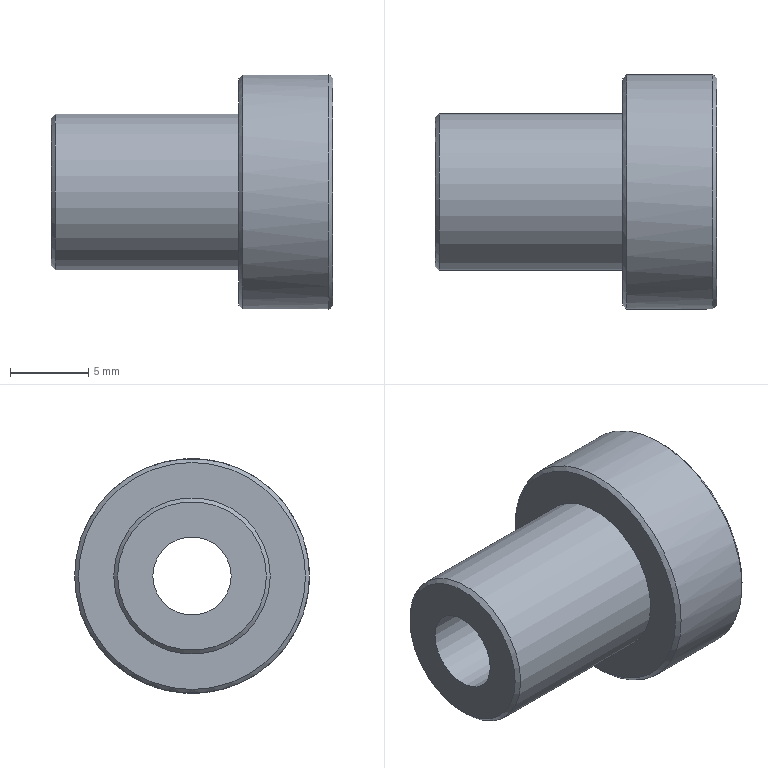Component | NX | PORT_1_2 | 1 solid | 9 faces | box 18 x 15 x 15 mm | volume 1645 mm3 | plane 3 | cylinder 3 | cone 3 | commonest cylinder face diameters 10 x1 15 x1 5 x1
STEP:
#1=CARTESIAN_POINT('',(0.,0.,0.));
#2=DIRECTION('',(0.,0.,1.));
#3=DIRECTION('',(1.,0.,0.));
#4=AXIS2_PLACEMENT_3D('',#1,#2,#3);
#5=CARTESIAN_POINT('',(-69.,-39.25,41.));
#6=VERTEX_POINT('',#5);
#7=CARTESIAN_POINT('',(-69.,-34.25,41.));
#8=VERTEX_POINT('',#7);
#9=CARTESIAN_POINT('',(-69.,-36.75,41.));
#10=DIRECTION('',(1.,0.,0.));
#11=DIRECTION('',(0.,-1.,0.));
#12=AXIS2_PLACEMENT_3D('',#9,#10,#11);
#13=CIRCLE('',#12,2.5);
#14=CARTESIAN_POINT('',(-69.,-36.75,41.));
#15=DIRECTION('',(-1.,0.,0.));
#16=DIRECTION('',(0.,-1.,0.));
#17=AXIS2_PLACEMENT_3D('',#14,#15,#16);
#18=PLANE('',#17);
#19=CARTESIAN_POINT('',(2.5,0.));
#20=CARTESIAN_POINT('',(2.5,-4.33));
#21=CARTESIAN_POINT('',(-1.25,-2.165));
#22=CARTESIAN_POINT('',(-5.,-0.));
#23=CARTESIAN_POINT('',(-1.25,2.165));
#24=CARTESIAN_POINT('',(2.5,4.33));
#25=CARTESIAN_POINT('',(2.5,0.));
#26=(BOUNDED_CURVE()B_SPLINE_CURVE(2,(#19,#20,#21,#22,#23,#24,#25),.UNSPECIFIED.,.T.,.F.)B_SPLINE_CURVE_WITH_KNOTS((1,2,2,2,2,1),(-2.094,0.,2.094,4.189,6.283,8.378),.UNSPECIFIED.)CURVE()GEOMETRIC_REPRESENTATION_ITEM()RATIONAL_B_SPLINE_CURVE((1.,0.5,1.,0.5,1.,0.5,1.))REPRESENTATION_ITEM(''));
#27=(GEOMETRIC_REPRESENTATION_CONTEXT(2)PARAMETRIC_REPRESENTATION_CONTEXT()REPRESENTATION_CONTEXT('',''));
#28=DEFINITIONAL_REPRESENTATION('',(#26),#27);
#29=PCURVE('',#18,#28);
#30=CARTESIAN_POINT('',(-76.,-36.75,41.));
#31=DIRECTION('',(1.,0.,0.));
#32=DIRECTION('',(0.,1.,0.));
#33=AXIS2_PLACEMENT_3D('',#30,#31,#32);
#34=CYLINDRICAL_SURFACE('',#33,2.5);
#35=CARTESIAN_POINT('',(3.142,7.));
#36=DIRECTION('',(1.,0.));
#37=VECTOR('',#36,1.);
#38=LINE('',#35,#37);
#39=(GEOMETRIC_REPRESENTATION_CONTEXT(2)PARAMETRIC_REPRESENTATION_CONTEXT()REPRESENTATION_CONTEXT('',''));
#40=DEFINITIONAL_REPRESENTATION('',(#38),#39);
#41=PCURVE('',#34,#40);
#42=SURFACE_CURVE('',#13,(#29,#41),.PCURVE_S1.);
#43=EDGE_CURVE('',#6,#8,#42,.T.);
#44=ORIENTED_EDGE('',*,*,#43,.T.);
#45=CARTESIAN_POINT('',(-69.,-36.75,41.));
#46=DIRECTION('',(1.,0.,0.));
#47=DIRECTION('',(0.,-1.,0.));
#48=AXIS2_PLACEMENT_3D('',#45,#46,#47);
#49=CIRCLE('',#48,2.5);
#50=CARTESIAN_POINT('',(2.5,0.));
#51=CARTESIAN_POINT('',(2.5,-4.33));
#52=CARTESIAN_POINT('',(-1.25,-2.165));
#53=CARTESIAN_POINT('',(-5.,-0.));
#54=CARTESIAN_POINT('',(-1.25,2.165));
#55=CARTESIAN_POINT('',(2.5,4.33));
#56=CARTESIAN_POINT('',(2.5,0.));
#57=(BOUNDED_CURVE()B_SPLINE_CURVE(2,(#50,#51,#52,#53,#54,#55,#56),.UNSPECIFIED.,.T.,.F.)B_SPLINE_CURVE_WITH_KNOTS((1,2,2,2,2,1),(-2.094,0.,2.094,4.189,6.283,8.378),.UNSPECIFIED.)CURVE()GEOMETRIC_REPRESENTATION_ITEM()RATIONAL_B_SPLINE_CURVE((1.,0.5,1.,0.5,1.,0.5,1.))REPRESENTATION_ITEM(''));
#58=(GEOMETRIC_REPRESENTATION_CONTEXT(2)PARAMETRIC_REPRESENTATION_CONTEXT()REPRESENTATION_CONTEXT('',''));
#59=DEFINITIONAL_REPRESENTATION('',(#57),#58);
#60=PCURVE('',#18,#59);
#61=CARTESIAN_POINT('',(-3.142,7.));
#62=DIRECTION('',(1.,0.));
#63=VECTOR('',#62,1.);
#64=LINE('',#61,#63);
#65=(GEOMETRIC_REPRESENTATION_CONTEXT(2)PARAMETRIC_REPRESENTATION_CONTEXT()REPRESENTATION_CONTEXT('',''));
#66=DEFINITIONAL_REPRESENTATION('',(#64),#65);
#67=PCURVE('',#34,#66);
#68=SURFACE_CURVE('',#49,(#60,#67),.PCURVE_S1.);
#69=EDGE_CURVE('',#8,#6,#68,.T.);
#70=ORIENTED_EDGE('',*,*,#69,.T.);
#71=EDGE_LOOP('',(#44,#70));
#72=FACE_BOUND('',#71,.T.);
#73=CARTESIAN_POINT('',(-69.,-41.5,41.));
#74=VERTEX_POINT('',#73);
#75=CARTESIAN_POINT('',(-69.,-36.75,41.));
#76=DIRECTION('',(-1.,0.,0.));
#77=DIRECTION('',(0.,-1.,0.));
#78=AXIS2_PLACEMENT_3D('',#75,#76,#77);
#79=CIRCLE('',#78,4.75);
#80=CARTESIAN_POINT('',(0.,0.));
#81=DIRECTION('',(1.,0.));
#82=AXIS2_PLACEMENT_2D('',#80,#81);
#83=CIRCLE('',#82,4.75);
#84=(GEOMETRIC_REPRESENTATION_CONTEXT(2)PARAMETRIC_REPRESENTATION_CONTEXT()REPRESENTATION_CONTEXT('',''));
#85=DEFINITIONAL_REPRESENTATION('',(#83),#84);
#86=PCURVE('',#18,#85);
#87=CARTESIAN_POINT('',(-68.75,-36.75,41.));
#88=DIRECTION('',(1.,0.,0.));
#89=DIRECTION('',(0.,1.,0.));
#90=AXIS2_PLACEMENT_3D('',#87,#88,#89);
#91=CONICAL_SURFACE('',#90,5.,0.7854);
#92=CARTESIAN_POINT('',(9.425,-0.25));
#93=DIRECTION('',(-1.,0.));
#94=VECTOR('',#93,1.);
#95=LINE('',#92,#94);
#96=(GEOMETRIC_REPRESENTATION_CONTEXT(2)PARAMETRIC_REPRESENTATION_CONTEXT()REPRESENTATION_CONTEXT('',''));
#97=DEFINITIONAL_REPRESENTATION('',(#95),#96);
#98=PCURVE('',#91,#97);
#99=SURFACE_CURVE('',#79,(#86,#98),.PCURVE_S1.);
#100=EDGE_CURVE('',#74,#74,#99,.T.);
#101=ORIENTED_EDGE('',*,*,#100,.T.);
#102=EDGE_LOOP('',(#101));
#103=FACE_BOUND('',#102,.T.);
#104=ADVANCED_FACE('',(#72,#103),#18,.T.);
#105=CARTESIAN_POINT('',(-68.75,-41.75,41.));
#106=VERTEX_POINT('',#105);
#107=CARTESIAN_POINT('',(-68.75,-31.75,41.));
#108=VERTEX_POINT('',#107);
#109=CARTESIAN_POINT('',(-68.75,-36.75,41.));
#110=DIRECTION('',(1.,0.,0.));
#111=DIRECTION('',(0.,-1.,0.));
#112=AXIS2_PLACEMENT_3D('',#109,#110,#111);
#113=CIRCLE('',#112,5.);
#114=CARTESIAN_POINT('',(-69.,-36.75,41.));
#115=DIRECTION('',(1.,0.,0.));
#116=DIRECTION('',(0.,1.,0.));
#117=AXIS2_PLACEMENT_3D('',#114,#115,#116);
#118=CYLINDRICAL_SURFACE('',#117,5.);
#119=CARTESIAN_POINT('',(3.142,0.25));
#120=DIRECTION('',(1.,0.));
#121=VECTOR('',#120,1.);
#122=LINE('',#119,#121);
#123=(GEOMETRIC_REPRESENTATION_CONTEXT(2)PARAMETRIC_REPRESENTATION_CONTEXT()REPRESENTATION_CONTEXT('',''));
#124=DEFINITIONAL_REPRESENTATION('',(#122),#123);
#125=PCURVE('',#118,#124);
#126=CARTESIAN_POINT('',(3.142,0.));
#127=DIRECTION('',(1.,0.));
#128=VECTOR('',#127,1.);
#129=LINE('',#126,#128);
#130=(GEOMETRIC_REPRESENTATION_CONTEXT(2)PARAMETRIC_REPRESENTATION_CONTEXT()REPRESENTATION_CONTEXT('',''));
#131=DEFINITIONAL_REPRESENTATION('',(#129),#130);
#132=PCURVE('',#91,#131);
#133=SURFACE_CURVE('',#113,(#125,#132),.PCURVE_S1.);
#134=EDGE_CURVE('',#106,#108,#133,.T.);
#135=ORIENTED_EDGE('',*,*,#134,.T.);
#136=CARTESIAN_POINT('',(-57.,-31.75,41.));
#137=VERTEX_POINT('',#136);
#138=CARTESIAN_POINT('',(-68.75,-31.75,41.));
#139=CARTESIAN_POINT('',(-57.,-31.75,41.));
#140=B_SPLINE_CURVE_WITH_KNOTS('',1,(#138,#139),.UNSPECIFIED.,.F.,.F.,(2,2),(0.25,12.),.PIECEWISE_BEZIER_KNOTS.);
#141=CARTESIAN_POINT('',(6.283,0.));
#142=DIRECTION('',(0.,1.));
#143=VECTOR('',#142,1.);
#144=LINE('',#141,#143);
#145=(GEOMETRIC_REPRESENTATION_CONTEXT(2)PARAMETRIC_REPRESENTATION_CONTEXT()REPRESENTATION_CONTEXT('',''));
#146=DEFINITIONAL_REPRESENTATION('',(#144),#145);
#147=PCURVE('',#118,#146);
#148=CARTESIAN_POINT('',(0.,0.));
#149=DIRECTION('',(0.,1.));
#150=VECTOR('',#149,1.);
#151=LINE('',#148,#150);
#152=(GEOMETRIC_REPRESENTATION_CONTEXT(2)PARAMETRIC_REPRESENTATION_CONTEXT()REPRESENTATION_CONTEXT('',''));
#153=DEFINITIONAL_REPRESENTATION('',(#151),#152);
#154=PCURVE('',#118,#153);
#155=SEAM_CURVE('',#140,(#147,#154),.PCURVE_S1.);
#156=EDGE_CURVE('',#108,#137,#155,.T.);
#157=ORIENTED_EDGE('',*,*,#156,.T.);
#158=CARTESIAN_POINT('',(-57.,-36.75,41.));
#159=DIRECTION('',(-1.,0.,0.));
#160=DIRECTION('',(0.,1.,0.));
#161=AXIS2_PLACEMENT_3D('',#158,#159,#160);
#162=CIRCLE('',#161,5.);
#163=CARTESIAN_POINT('',(6.283,12.));
#164=DIRECTION('',(-1.,0.));
#165=VECTOR('',#164,1.);
#166=LINE('',#163,#165);
#167=(GEOMETRIC_REPRESENTATION_CONTEXT(2)PARAMETRIC_REPRESENTATION_CONTEXT()REPRESENTATION_CONTEXT('',''));
#168=DEFINITIONAL_REPRESENTATION('',(#166),#167);
#169=PCURVE('',#118,#168);
#170=CARTESIAN_POINT('',(-57.,-36.75,41.));
#171=DIRECTION('',(-1.,0.,0.));
#172=DIRECTION('',(0.,-1.,0.));
#173=AXIS2_PLACEMENT_3D('',#170,#171,#172);
#174=PLANE('',#173);
#175=CARTESIAN_POINT('',(0.,0.));
#176=DIRECTION('',(-1.,0.));
#177=AXIS2_PLACEMENT_2D('',#175,#176);
#178=CIRCLE('',#177,5.);
#179=(GEOMETRIC_REPRESENTATION_CONTEXT(2)PARAMETRIC_REPRESENTATION_CONTEXT()REPRESENTATION_CONTEXT('',''));
#180=DEFINITIONAL_REPRESENTATION('',(#178),#179);
#181=PCURVE('',#174,#180);
#182=SURFACE_CURVE('',#162,(#169,#181),.PCURVE_S1.);
#183=EDGE_CURVE('',#137,#137,#182,.T.);
#184=ORIENTED_EDGE('',*,*,#183,.T.);
#185=ORIENTED_EDGE('',*,*,#156,.F.);
#186=CARTESIAN_POINT('',(-68.75,-36.75,41.));
#187=DIRECTION('',(1.,0.,0.));
#188=DIRECTION('',(0.,-1.,0.));
#189=AXIS2_PLACEMENT_3D('',#186,#187,#188);
#190=CIRCLE('',#189,5.);
#191=CARTESIAN_POINT('',(-3.142,0.25));
#192=DIRECTION('',(1.,0.));
#193=VECTOR('',#192,1.);
#194=LINE('',#191,#193);
#195=(GEOMETRIC_REPRESENTATION_CONTEXT(2)PARAMETRIC_REPRESENTATION_CONTEXT()REPRESENTATION_CONTEXT('',''));
#196=DEFINITIONAL_REPRESENTATION('',(#194),#195);
#197=PCURVE('',#118,#196);
#198=CARTESIAN_POINT('',(3.142,0.));
#199=DIRECTION('',(1.,0.));
#200=VECTOR('',#199,1.);
#201=LINE('',#198,#200);
#202=(GEOMETRIC_REPRESENTATION_CONTEXT(2)PARAMETRIC_REPRESENTATION_CONTEXT()REPRESENTATION_CONTEXT('',''));
#203=DEFINITIONAL_REPRESENTATION('',(#201),#202);
#204=PCURVE('',#91,#203);
#205=SURFACE_CURVE('',#190,(#197,#204),.PCURVE_S1.);
#206=EDGE_CURVE('',#108,#106,#205,.T.);
#207=ORIENTED_EDGE('',*,*,#206,.T.);
#208=EDGE_LOOP('',(#135,#157,#184,#185,#207));
#209=FACE_BOUND('',#208,.T.);
#210=ADVANCED_FACE('',(#209),#118,.T.);
#211=CARTESIAN_POINT('',(-51.,-34.25,41.));
#212=VERTEX_POINT('',#211);
#213=CARTESIAN_POINT('',(-51.,-36.75,41.));
#214=DIRECTION('',(-1.,0.,0.));
#215=DIRECTION('',(0.,1.,0.));
#216=AXIS2_PLACEMENT_3D('',#213,#214,#215);
#217=CIRCLE('',#216,2.5);
#218=CARTESIAN_POINT('',(-51.,-36.75,41.));
#219=DIRECTION('',(1.,0.,0.));
#220=DIRECTION('',(0.,1.,0.));
#221=AXIS2_PLACEMENT_3D('',#218,#219,#220);
#222=PLANE('',#221);
#223=CARTESIAN_POINT('',(2.5,0.));
#224=CARTESIAN_POINT('',(2.5,-4.33));
#225=CARTESIAN_POINT('',(-1.25,-2.165));
#226=CARTESIAN_POINT('',(-5.,-0.));
#227=CARTESIAN_POINT('',(-1.25,2.165));
#228=CARTESIAN_POINT('',(2.5,4.33));
#229=CARTESIAN_POINT('',(2.5,0.));
#230=(BOUNDED_CURVE()B_SPLINE_CURVE(2,(#223,#224,#225,#226,#227,#228,#229),.UNSPECIFIED.,.T.,.F.)B_SPLINE_CURVE_WITH_KNOTS((1,2,2,2,2,1),(-2.094,0.,2.094,4.189,6.283,8.378),.UNSPECIFIED.)CURVE()GEOMETRIC_REPRESENTATION_ITEM()RATIONAL_B_SPLINE_CURVE((1.,0.5,1.,0.5,1.,0.5,1.))REPRESENTATION_ITEM(''));
#231=(GEOMETRIC_REPRESENTATION_CONTEXT(2)PARAMETRIC_REPRESENTATION_CONTEXT()REPRESENTATION_CONTEXT('',''));
#232=DEFINITIONAL_REPRESENTATION('',(#230),#231);
#233=PCURVE('',#222,#232);
#234=CARTESIAN_POINT('',(6.283,25.));
#235=DIRECTION('',(-1.,0.));
#236=VECTOR('',#235,1.);
#237=LINE('',#234,#236);
#238=(GEOMETRIC_REPRESENTATION_CONTEXT(2)PARAMETRIC_REPRESENTATION_CONTEXT()REPRESENTATION_CONTEXT('',''));
#239=DEFINITIONAL_REPRESENTATION('',(#237),#238);
#240=PCURVE('',#34,#239);
#241=SURFACE_CURVE('',#217,(#233,#240),.PCURVE_S1.);
#242=EDGE_CURVE('',#212,#212,#241,.T.);
#243=ORIENTED_EDGE('',*,*,#242,.T.);
#244=EDGE_LOOP('',(#243));
#245=FACE_BOUND('',#244,.T.);
#246=CARTESIAN_POINT('',(-51.,-29.5,41.));
#247=VERTEX_POINT('',#246);
#248=CARTESIAN_POINT('',(-51.,-36.75,41.));
#249=DIRECTION('',(1.,0.,0.));
#250=DIRECTION('',(0.,1.,0.));
#251=AXIS2_PLACEMENT_3D('',#248,#249,#250);
#252=CIRCLE('',#251,7.25);
#253=CARTESIAN_POINT('',(0.,0.));
#254=DIRECTION('',(1.,0.));
#255=AXIS2_PLACEMENT_2D('',#253,#254);
#256=CIRCLE('',#255,7.25);
#257=(GEOMETRIC_REPRESENTATION_CONTEXT(2)PARAMETRIC_REPRESENTATION_CONTEXT()REPRESENTATION_CONTEXT('',''));
#258=DEFINITIONAL_REPRESENTATION('',(#256),#257);
#259=PCURVE('',#222,#258);
#260=CARTESIAN_POINT('',(-51.,-36.75,41.));
#261=DIRECTION('',(-1.,0.,0.));
#262=DIRECTION('',(0.,-1.,0.));
#263=AXIS2_PLACEMENT_3D('',#260,#261,#262);
#264=CONICAL_SURFACE('',#263,7.25,0.7854);
#265=CARTESIAN_POINT('',(9.425,0.));
#266=DIRECTION('',(-1.,0.));
#267=VECTOR('',#266,1.);
#268=LINE('',#265,#267);
#269=(GEOMETRIC_REPRESENTATION_CONTEXT(2)PARAMETRIC_REPRESENTATION_CONTEXT()REPRESENTATION_CONTEXT('',''));
#270=DEFINITIONAL_REPRESENTATION('',(#268),#269);
#271=PCURVE('',#264,#270);
#272=SURFACE_CURVE('',#252,(#259,#271),.PCURVE_S1.);
#273=EDGE_CURVE('',#247,#247,#272,.T.);
#274=ORIENTED_EDGE('',*,*,#273,.T.);
#275=EDGE_LOOP('',(#274));
#276=FACE_BOUND('',#275,.T.);
#277=ADVANCED_FACE('',(#245,#276),#222,.T.);
#278=CARTESIAN_POINT('',(-57.,-44.,41.));
#279=VERTEX_POINT('',#278);
#280=CARTESIAN_POINT('',(-57.,-36.75,41.));
#281=DIRECTION('',(-1.,0.,0.));
#282=DIRECTION('',(0.,-1.,0.));
#283=AXIS2_PLACEMENT_3D('',#280,#281,#282);
#284=CIRCLE('',#283,7.25);
#285=CARTESIAN_POINT('',(0.,0.));
#286=DIRECTION('',(1.,0.));
#287=AXIS2_PLACEMENT_2D('',#285,#286);
#288=CIRCLE('',#287,7.25);
#289=(GEOMETRIC_REPRESENTATION_CONTEXT(2)PARAMETRIC_REPRESENTATION_CONTEXT()REPRESENTATION_CONTEXT('',''));
#290=DEFINITIONAL_REPRESENTATION('',(#288),#289);
#291=PCURVE('',#174,#290);
#292=CARTESIAN_POINT('',(-56.75,-36.75,41.));
#293=DIRECTION('',(1.,0.,0.));
#294=DIRECTION('',(0.,1.,0.));
#295=AXIS2_PLACEMENT_3D('',#292,#293,#294);
#296=CONICAL_SURFACE('',#295,7.5,0.7854);
#297=CARTESIAN_POINT('',(9.425,-0.25));
#298=DIRECTION('',(-1.,0.));
#299=VECTOR('',#298,1.);
#300=LINE('',#297,#299);
#301=(GEOMETRIC_REPRESENTATION_CONTEXT(2)PARAMETRIC_REPRESENTATION_CONTEXT()REPRESENTATION_CONTEXT('',''));
#302=DEFINITIONAL_REPRESENTATION('',(#300),#301);
#303=PCURVE('',#296,#302);
#304=SURFACE_CURVE('',#284,(#291,#303),.PCURVE_S1.);
#305=EDGE_CURVE('',#279,#279,#304,.T.);
#306=ORIENTED_EDGE('',*,*,#305,.T.);
#307=EDGE_LOOP('',(#306));
#308=FACE_BOUND('',#307,.T.);
#309=ORIENTED_EDGE('',*,*,#183,.F.);
#310=EDGE_LOOP('',(#309));
#311=FACE_BOUND('',#310,.T.);
#312=ADVANCED_FACE('',(#308,#311),#174,.T.);
#313=CARTESIAN_POINT('',(-56.75,-44.25,41.));
#314=VERTEX_POINT('',#313);
#315=CARTESIAN_POINT('',(-56.75,-29.25,41.));
#316=VERTEX_POINT('',#315);
#317=CARTESIAN_POINT('',(-56.75,-36.75,41.));
#318=DIRECTION('',(1.,0.,0.));
#319=DIRECTION('',(0.,-1.,0.));
#320=AXIS2_PLACEMENT_3D('',#317,#318,#319);
#321=CIRCLE('',#320,7.5);
#322=CARTESIAN_POINT('',(-57.,-36.75,41.));
#323=DIRECTION('',(1.,0.,0.));
#324=DIRECTION('',(0.,1.,0.));
#325=AXIS2_PLACEMENT_3D('',#322,#323,#324);
#326=CYLINDRICAL_SURFACE('',#325,7.5);
#327=CARTESIAN_POINT('',(3.142,0.25));
#328=DIRECTION('',(1.,0.));
#329=VECTOR('',#328,1.);
#330=LINE('',#327,#329);
#331=(GEOMETRIC_REPRESENTATION_CONTEXT(2)PARAMETRIC_REPRESENTATION_CONTEXT()REPRESENTATION_CONTEXT('',''));
#332=DEFINITIONAL_REPRESENTATION('',(#330),#331);
#333=PCURVE('',#326,#332);
#334=CARTESIAN_POINT('',(3.142,0.));
#335=DIRECTION('',(1.,0.));
#336=VECTOR('',#335,1.);
#337=LINE('',#334,#336);
#338=(GEOMETRIC_REPRESENTATION_CONTEXT(2)PARAMETRIC_REPRESENTATION_CONTEXT()REPRESENTATION_CONTEXT('',''));
#339=DEFINITIONAL_REPRESENTATION('',(#337),#338);
#340=PCURVE('',#296,#339);
#341=SURFACE_CURVE('',#321,(#333,#340),.PCURVE_S1.);
#342=EDGE_CURVE('',#314,#316,#341,.T.);
#343=ORIENTED_EDGE('',*,*,#342,.T.);
#344=CARTESIAN_POINT('',(-51.25,-29.25,41.));
#345=VERTEX_POINT('',#344);
#346=CARTESIAN_POINT('',(-56.75,-29.25,41.));
#347=CARTESIAN_POINT('',(-51.25,-29.25,41.));
#348=B_SPLINE_CURVE_WITH_KNOTS('',1,(#346,#347),.UNSPECIFIED.,.F.,.F.,(2,2),(0.25,5.75),.PIECEWISE_BEZIER_KNOTS.);
#349=CARTESIAN_POINT('',(6.283,0.));
#350=DIRECTION('',(0.,1.));
#351=VECTOR('',#350,1.);
#352=LINE('',#349,#351);
#353=(GEOMETRIC_REPRESENTATION_CONTEXT(2)PARAMETRIC_REPRESENTATION_CONTEXT()REPRESENTATION_CONTEXT('',''));
#354=DEFINITIONAL_REPRESENTATION('',(#352),#353);
#355=PCURVE('',#326,#354);
#356=CARTESIAN_POINT('',(0.,0.));
#357=DIRECTION('',(0.,1.));
#358=VECTOR('',#357,1.);
#359=LINE('',#356,#358);
#360=(GEOMETRIC_REPRESENTATION_CONTEXT(2)PARAMETRIC_REPRESENTATION_CONTEXT()REPRESENTATION_CONTEXT('',''));
#361=DEFINITIONAL_REPRESENTATION('',(#359),#360);
#362=PCURVE('',#326,#361);
#363=SEAM_CURVE('',#348,(#355,#362),.PCURVE_S1.);
#364=EDGE_CURVE('',#316,#345,#363,.T.);
#365=ORIENTED_EDGE('',*,*,#364,.T.);
#366=CARTESIAN_POINT('',(-51.25,-36.75,41.));
#367=DIRECTION('',(-1.,0.,0.));
#368=DIRECTION('',(0.,1.,0.));
#369=AXIS2_PLACEMENT_3D('',#366,#367,#368);
#370=CIRCLE('',#369,7.5);
#371=CARTESIAN_POINT('',(6.283,5.75));
#372=DIRECTION('',(-1.,0.));
#373=VECTOR('',#372,1.);
#374=LINE('',#371,#373);
#375=(GEOMETRIC_REPRESENTATION_CONTEXT(2)PARAMETRIC_REPRESENTATION_CONTEXT()REPRESENTATION_CONTEXT('',''));
#376=DEFINITIONAL_REPRESENTATION('',(#374),#375);
#377=PCURVE('',#326,#376);
#378=CARTESIAN_POINT('',(3.142,0.25));
#379=DIRECTION('',(1.,0.));
#380=VECTOR('',#379,1.);
#381=LINE('',#378,#380);
#382=(GEOMETRIC_REPRESENTATION_CONTEXT(2)PARAMETRIC_REPRESENTATION_CONTEXT()REPRESENTATION_CONTEXT('',''));
#383=DEFINITIONAL_REPRESENTATION('',(#381),#382);
#384=PCURVE('',#264,#383);
#385=SURFACE_CURVE('',#370,(#377,#384),.PCURVE_S1.);
#386=EDGE_CURVE('',#345,#345,#385,.T.);
#387=ORIENTED_EDGE('',*,*,#386,.T.);
#388=ORIENTED_EDGE('',*,*,#364,.F.);
#389=CARTESIAN_POINT('',(-56.75,-36.75,41.));
#390=DIRECTION('',(1.,0.,0.));
#391=DIRECTION('',(0.,-1.,0.));
#392=AXIS2_PLACEMENT_3D('',#389,#390,#391);
#393=CIRCLE('',#392,7.5);
#394=CARTESIAN_POINT('',(-3.142,0.25));
#395=DIRECTION('',(1.,0.));
#396=VECTOR('',#395,1.);
#397=LINE('',#394,#396);
#398=(GEOMETRIC_REPRESENTATION_CONTEXT(2)PARAMETRIC_REPRESENTATION_CONTEXT()REPRESENTATION_CONTEXT('',''));
#399=DEFINITIONAL_REPRESENTATION('',(#397),#398);
#400=PCURVE('',#326,#399);
#401=CARTESIAN_POINT('',(3.142,0.));
#402=DIRECTION('',(1.,0.));
#403=VECTOR('',#402,1.);
#404=LINE('',#401,#403);
#405=(GEOMETRIC_REPRESENTATION_CONTEXT(2)PARAMETRIC_REPRESENTATION_CONTEXT()REPRESENTATION_CONTEXT('',''));
#406=DEFINITIONAL_REPRESENTATION('',(#404),#405);
#407=PCURVE('',#296,#406);
#408=SURFACE_CURVE('',#393,(#400,#407),.PCURVE_S1.);
#409=EDGE_CURVE('',#316,#314,#408,.T.);
#410=ORIENTED_EDGE('',*,*,#409,.T.);
#411=EDGE_LOOP('',(#343,#365,#387,#388,#410));
#412=FACE_BOUND('',#411,.T.);
#413=ADVANCED_FACE('',(#412),#326,.T.);
#414=ORIENTED_EDGE('',*,*,#305,.F.);
#415=CARTESIAN_POINT('',(-57.,-44.,41.));
#416=CARTESIAN_POINT('',(-56.75,-44.25,41.));
#417=B_SPLINE_CURVE_WITH_KNOTS('',1,(#415,#416),.UNSPECIFIED.,.F.,.F.,(2,2),(-0.3536,0.),.PIECEWISE_BEZIER_KNOTS.);
#418=CARTESIAN_POINT('',(9.425,0.));
#419=DIRECTION('',(0.,1.));
#420=VECTOR('',#419,1.);
#421=LINE('',#418,#420);
#422=(GEOMETRIC_REPRESENTATION_CONTEXT(2)PARAMETRIC_REPRESENTATION_CONTEXT()REPRESENTATION_CONTEXT('',''));
#423=DEFINITIONAL_REPRESENTATION('',(#421),#422);
#424=PCURVE('',#296,#423);
#425=CARTESIAN_POINT('',(3.142,0.));
#426=DIRECTION('',(0.,1.));
#427=VECTOR('',#426,1.);
#428=LINE('',#425,#427);
#429=(GEOMETRIC_REPRESENTATION_CONTEXT(2)PARAMETRIC_REPRESENTATION_CONTEXT()REPRESENTATION_CONTEXT('',''));
#430=DEFINITIONAL_REPRESENTATION('',(#428),#429);
#431=PCURVE('',#296,#430);
#432=SEAM_CURVE('',#417,(#424,#431),.PCURVE_S1.);
#433=EDGE_CURVE('',#279,#314,#432,.T.);
#434=ORIENTED_EDGE('',*,*,#433,.T.);
#435=ORIENTED_EDGE('',*,*,#409,.F.);
#436=ORIENTED_EDGE('',*,*,#342,.F.);
#437=ORIENTED_EDGE('',*,*,#433,.F.);
#438=EDGE_LOOP('',(#414,#434,#435,#436,#437));
#439=FACE_BOUND('',#438,.T.);
#440=ADVANCED_FACE('',(#439),#296,.T.);
#441=ORIENTED_EDGE('',*,*,#386,.F.);
#442=CARTESIAN_POINT('',(-51.,-29.5,41.));
#443=CARTESIAN_POINT('',(-51.25,-29.25,41.));
#444=B_SPLINE_CURVE_WITH_KNOTS('',1,(#442,#443),.UNSPECIFIED.,.F.,.F.,(2,2),(0.,0.3536),.PIECEWISE_BEZIER_KNOTS.);
#445=CARTESIAN_POINT('',(3.142,0.));
#446=DIRECTION('',(0.,1.));
#447=VECTOR('',#446,1.);
#448=LINE('',#445,#447);
#449=(GEOMETRIC_REPRESENTATION_CONTEXT(2)PARAMETRIC_REPRESENTATION_CONTEXT()REPRESENTATION_CONTEXT('',''));
#450=DEFINITIONAL_REPRESENTATION('',(#448),#449);
#451=PCURVE('',#264,#450);
#452=CARTESIAN_POINT('',(9.425,0.));
#453=DIRECTION('',(0.,1.));
#454=VECTOR('',#453,1.);
#455=LINE('',#452,#454);
#456=(GEOMETRIC_REPRESENTATION_CONTEXT(2)PARAMETRIC_REPRESENTATION_CONTEXT()REPRESENTATION_CONTEXT('',''));
#457=DEFINITIONAL_REPRESENTATION('',(#455),#456);
#458=PCURVE('',#264,#457);
#459=SEAM_CURVE('',#444,(#451,#458),.PCURVE_S1.);
#460=EDGE_CURVE('',#247,#345,#459,.T.);
#461=ORIENTED_EDGE('',*,*,#460,.F.);
#462=ORIENTED_EDGE('',*,*,#273,.F.);
#463=ORIENTED_EDGE('',*,*,#460,.T.);
#464=EDGE_LOOP('',(#441,#461,#462,#463));
#465=FACE_BOUND('',#464,.T.);
#466=ADVANCED_FACE('',(#465),#264,.T.);
#467=ORIENTED_EDGE('',*,*,#100,.F.);
#468=CARTESIAN_POINT('',(-69.,-41.5,41.));
#469=CARTESIAN_POINT('',(-68.75,-41.75,41.));
#470=B_SPLINE_CURVE_WITH_KNOTS('',1,(#468,#469),.UNSPECIFIED.,.F.,.F.,(2,2),(-0.3536,0.),.PIECEWISE_BEZIER_KNOTS.);
#471=CARTESIAN_POINT('',(9.425,0.));
#472=DIRECTION('',(0.,1.));
#473=VECTOR('',#472,1.);
#474=LINE('',#471,#473);
#475=(GEOMETRIC_REPRESENTATION_CONTEXT(2)PARAMETRIC_REPRESENTATION_CONTEXT()REPRESENTATION_CONTEXT('',''));
#476=DEFINITIONAL_REPRESENTATION('',(#474),#475);
#477=PCURVE('',#91,#476);
#478=CARTESIAN_POINT('',(3.142,0.));
#479=DIRECTION('',(0.,1.));
#480=VECTOR('',#479,1.);
#481=LINE('',#478,#480);
#482=(GEOMETRIC_REPRESENTATION_CONTEXT(2)PARAMETRIC_REPRESENTATION_CONTEXT()REPRESENTATION_CONTEXT('',''));
#483=DEFINITIONAL_REPRESENTATION('',(#481),#482);
#484=PCURVE('',#91,#483);
#485=SEAM_CURVE('',#470,(#477,#484),.PCURVE_S1.);
#486=EDGE_CURVE('',#74,#106,#485,.T.);
#487=ORIENTED_EDGE('',*,*,#486,.T.);
#488=ORIENTED_EDGE('',*,*,#206,.F.);
#489=ORIENTED_EDGE('',*,*,#134,.F.);
#490=ORIENTED_EDGE('',*,*,#486,.F.);
#491=EDGE_LOOP('',(#467,#487,#488,#489,#490));
#492=FACE_BOUND('',#491,.T.);
#493=ADVANCED_FACE('',(#492),#91,.T.);
#494=ORIENTED_EDGE('',*,*,#43,.T.);
#495=CARTESIAN_POINT('',(-69.,-34.25,41.));
#496=CARTESIAN_POINT('',(-51.,-34.25,41.));
#497=B_SPLINE_CURVE_WITH_KNOTS('',1,(#495,#496),.UNSPECIFIED.,.F.,.F.,(2,2),(7.,25.),.PIECEWISE_BEZIER_KNOTS.);
#498=CARTESIAN_POINT('',(6.283,0.));
#499=DIRECTION('',(0.,1.));
#500=VECTOR('',#499,1.);
#501=LINE('',#498,#500);
#502=(GEOMETRIC_REPRESENTATION_CONTEXT(2)PARAMETRIC_REPRESENTATION_CONTEXT()REPRESENTATION_CONTEXT('',''));
#503=DEFINITIONAL_REPRESENTATION('',(#501),#502);
#504=PCURVE('',#34,#503);
#505=CARTESIAN_POINT('',(0.,0.));
#506=DIRECTION('',(0.,1.));
#507=VECTOR('',#506,1.);
#508=LINE('',#505,#507);
#509=(GEOMETRIC_REPRESENTATION_CONTEXT(2)PARAMETRIC_REPRESENTATION_CONTEXT()REPRESENTATION_CONTEXT('',''));
#510=DEFINITIONAL_REPRESENTATION('',(#508),#509);
#511=PCURVE('',#34,#510);
#512=SEAM_CURVE('',#497,(#504,#511),.PCURVE_S1.);
#513=EDGE_CURVE('',#8,#212,#512,.T.);
#514=ORIENTED_EDGE('',*,*,#513,.T.);
#515=ORIENTED_EDGE('',*,*,#242,.T.);
#516=ORIENTED_EDGE('',*,*,#513,.F.);
#517=ORIENTED_EDGE('',*,*,#69,.T.);
#518=EDGE_LOOP('',(#494,#514,#515,#516,#517));
#519=FACE_BOUND('',#518,.F.);
#520=ADVANCED_FACE('',(#519),#34,.F.);
#521=CLOSED_SHELL('',(#104,#210,#277,#312,#413,#440,#466,#493,#520));
#522=MANIFOLD_SOLID_BREP('',#521);
#523=(LENGTH_UNIT()NAMED_UNIT(*)SI_UNIT(.MILLI.,.METRE.));
#524=UNCERTAINTY_MEASURE_WITH_UNIT(LENGTH_MEASURE(0.00001),#523,'','');
#525=(NAMED_UNIT(*)PLANE_ANGLE_UNIT()SI_UNIT($,.RADIAN.));
#526=(NAMED_UNIT(*)SI_UNIT($,.STERADIAN.)SOLID_ANGLE_UNIT());
#527=(GEOMETRIC_REPRESENTATION_CONTEXT(3)GLOBAL_UNCERTAINTY_ASSIGNED_CONTEXT((#524))GLOBAL_UNIT_ASSIGNED_CONTEXT((#523,#525,#526))REPRESENTATION_CONTEXT('',''));
#528=ADVANCED_BREP_SHAPE_REPRESENTATION('',(#4,#522),#527);